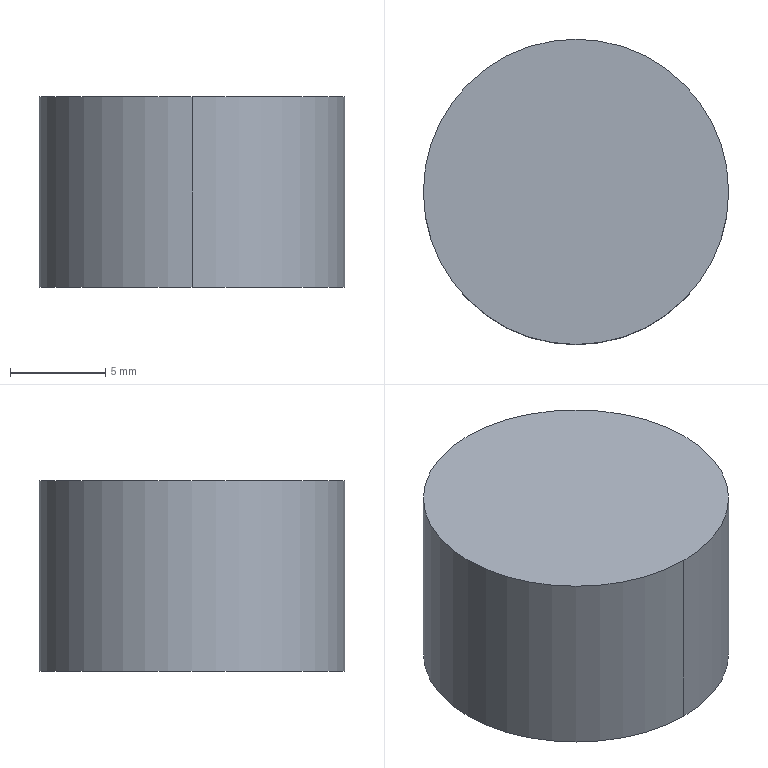Component | SolidWorks | JF21-80.1-1-3(_)-1-SOLID76-1 | 1 solid | 4 faces | box 16 x 16 x 10 mm | volume 2011 mm3 | cylinder 2 | plane 2 | commonest cylinder face diameters 16 x2
STEP:
#1=CARTESIAN_POINT('',(4.429,3.366,-9.449));
#2=VERTEX_POINT('',#1);
#3=CARTESIAN_POINT('',(4.429,2.736,-9.449));
#4=VERTEX_POINT('',#3);
#5=CARTESIAN_POINT('',(4.429,3.051,-9.449));
#6=DIRECTION('',(0.,0.,-1.));
#7=DIRECTION('',(0.,1.,0.));
#8=AXIS2_PLACEMENT_3D('',#5,#6,#7);
#9=CIRCLE('',#8,0.315);
#10=EDGE_CURVE('',#2,#4,#9,.T.);
#11=ORIENTED_EDGE('',*,*,#10,.T.);
#12=CARTESIAN_POINT('',(4.429,2.736,-9.843));
#13=VERTEX_POINT('',#12);
#14=CARTESIAN_POINT('',(4.429,2.736,-9.449));
#15=DIRECTION('',(0.,0.,-1.));
#16=VECTOR('',#15,39.37);
#17=LINE('',#14,#16);
#18=EDGE_CURVE('',#4,#13,#17,.T.);
#19=ORIENTED_EDGE('',*,*,#18,.T.);
#20=CARTESIAN_POINT('',(4.429,3.366,-9.843));
#21=VERTEX_POINT('',#20);
#22=CARTESIAN_POINT('',(4.429,3.051,-9.843));
#23=DIRECTION('',(0.,0.,-1.));
#24=DIRECTION('',(0.,1.,0.));
#25=AXIS2_PLACEMENT_3D('',#22,#23,#24);
#26=CIRCLE('',#25,0.315);
#27=EDGE_CURVE('',#21,#13,#26,.T.);
#28=ORIENTED_EDGE('',*,*,#27,.F.);
#29=CARTESIAN_POINT('',(4.429,3.366,-9.449));
#30=DIRECTION('',(0.,0.,-1.));
#31=VECTOR('',#30,39.37);
#32=LINE('',#29,#31);
#33=EDGE_CURVE('',#2,#21,#32,.T.);
#34=ORIENTED_EDGE('',*,*,#33,.F.);
#35=EDGE_LOOP('',(#11,#19,#28,#34));
#36=FACE_OUTER_BOUND('',#35,.T.);
#37=CARTESIAN_POINT('',(4.429,3.051,-9.449));
#38=DIRECTION('',(0.,0.,-1.));
#39=DIRECTION('',(0.,-1.,0.));
#40=AXIS2_PLACEMENT_3D('',#37,#38,#39);
#41=CYLINDRICAL_SURFACE('',#40,0.315);
#42=ADVANCED_FACE('',(#36),#41,.T.);
#43=ORIENTED_EDGE('',*,*,#18,.F.);
#44=CARTESIAN_POINT('',(4.429,3.051,-9.449));
#45=DIRECTION('',(0.,0.,-1.));
#46=DIRECTION('',(0.,1.,0.));
#47=AXIS2_PLACEMENT_3D('',#44,#45,#46);
#48=CIRCLE('',#47,0.315);
#49=EDGE_CURVE('',#4,#2,#48,.T.);
#50=ORIENTED_EDGE('',*,*,#49,.T.);
#51=ORIENTED_EDGE('',*,*,#33,.T.);
#52=CARTESIAN_POINT('',(4.429,3.051,-9.843));
#53=DIRECTION('',(0.,0.,-1.));
#54=DIRECTION('',(0.,1.,0.));
#55=AXIS2_PLACEMENT_3D('',#52,#53,#54);
#56=CIRCLE('',#55,0.315);
#57=EDGE_CURVE('',#13,#21,#56,.T.);
#58=ORIENTED_EDGE('',*,*,#57,.F.);
#59=EDGE_LOOP('',(#43,#50,#51,#58));
#60=FACE_OUTER_BOUND('',#59,.T.);
#61=CARTESIAN_POINT('',(4.429,3.051,-9.449));
#62=DIRECTION('',(0.,0.,-1.));
#63=DIRECTION('',(0.,-1.,0.));
#64=AXIS2_PLACEMENT_3D('',#61,#62,#63);
#65=CYLINDRICAL_SURFACE('',#64,0.315);
#66=ADVANCED_FACE('',(#60),#65,.T.);
#67=ORIENTED_EDGE('',*,*,#10,.F.);
#68=ORIENTED_EDGE('',*,*,#49,.F.);
#69=EDGE_LOOP('',(#67,#68));
#70=FACE_OUTER_BOUND('',#69,.T.);
#71=CARTESIAN_POINT('',(4.429,3.051,-9.449));
#72=DIRECTION('',(0.,0.,-1.));
#73=DIRECTION('',(0.,-1.,-0.));
#74=AXIS2_PLACEMENT_3D('',#71,#72,#73);
#75=PLANE('',#74);
#76=ADVANCED_FACE('',(#70),#75,.F.);
#77=ORIENTED_EDGE('',*,*,#27,.T.);
#78=ORIENTED_EDGE('',*,*,#57,.T.);
#79=EDGE_LOOP('',(#77,#78));
#80=FACE_OUTER_BOUND('',#79,.T.);
#81=CARTESIAN_POINT('',(4.429,3.051,-9.843));
#82=DIRECTION('',(0.,0.,-1.));
#83=DIRECTION('',(0.,-1.,-0.));
#84=AXIS2_PLACEMENT_3D('',#81,#82,#83);
#85=PLANE('',#84);
#86=ADVANCED_FACE('',(#80),#85,.T.);
#87=CLOSED_SHELL('',(#42,#66,#76,#86));
#88=MANIFOLD_SOLID_BREP('',#87);
#89=CARTESIAN_POINT('',(0.,0.,0.));
#90=DIRECTION('',(0.,0.,1.));
#91=DIRECTION('',(1.,0.,0.));
#92=AXIS2_PLACEMENT_3D('',#89,#90,#91);
#93=(LENGTH_UNIT()NAMED_UNIT(*)SI_UNIT($,.METRE.));
#94=LENGTH_MEASURE_WITH_UNIT(LENGTH_MEASURE(0.0254),#93);
#95=DIMENSIONAL_EXPONENTS(1.,0.,0.,0.,0.,0.,0.);
#96=(CONVERSION_BASED_UNIT('',#94)LENGTH_UNIT()NAMED_UNIT(#95));
#97=UNCERTAINTY_MEASURE_WITH_UNIT(LENGTH_MEASURE(0.00001),#96,'','');
#98=(NAMED_UNIT(*)PLANE_ANGLE_UNIT()SI_UNIT($,.RADIAN.));
#99=(NAMED_UNIT(*)SI_UNIT($,.STERADIAN.)SOLID_ANGLE_UNIT());
#100=(GEOMETRIC_REPRESENTATION_CONTEXT(3)GLOBAL_UNCERTAINTY_ASSIGNED_CONTEXT((#97))GLOBAL_UNIT_ASSIGNED_CONTEXT((#96,#98,#99))REPRESENTATION_CONTEXT('',''));
#101=ADVANCED_BREP_SHAPE_REPRESENTATION('',(#88,#92),#100);
#102=COLOUR_RGB('',0.7922,0.8196,0.9333);
#103=FILL_AREA_STYLE_COLOUR('',#102);
#104=FILL_AREA_STYLE('',(#103));
#105=SURFACE_STYLE_FILL_AREA(#104);
#106=SURFACE_SIDE_STYLE('',(#105));
#107=SURFACE_STYLE_USAGE(.BOTH.,#106);
#108=PRESENTATION_STYLE_ASSIGNMENT((#107));
#109=STYLED_ITEM('',(#108),#88);
#110=(LENGTH_UNIT()NAMED_UNIT(*)SI_UNIT($,.METRE.));
#111=LENGTH_MEASURE_WITH_UNIT(LENGTH_MEASURE(0.0254),#110);
#112=DIMENSIONAL_EXPONENTS(1.,0.,0.,0.,0.,0.,0.);
#113=(CONVERSION_BASED_UNIT('',#111)LENGTH_UNIT()NAMED_UNIT(#112));
#114=UNCERTAINTY_MEASURE_WITH_UNIT(LENGTH_MEASURE(0.00001),#113,'','');
#115=(NAMED_UNIT(*)PLANE_ANGLE_UNIT()SI_UNIT($,.RADIAN.));
#116=(NAMED_UNIT(*)SI_UNIT($,.STERADIAN.)SOLID_ANGLE_UNIT());
#117=(GEOMETRIC_REPRESENTATION_CONTEXT(3)GLOBAL_UNCERTAINTY_ASSIGNED_CONTEXT((#114))GLOBAL_UNIT_ASSIGNED_CONTEXT((#113,#115,#116))REPRESENTATION_CONTEXT('',''));
#118=MECHANICAL_DESIGN_GEOMETRIC_PRESENTATION_REPRESENTATION('',(#109),#117);
#119=PRESENTATION_LAYER_ASSIGNMENT('','',(#109));